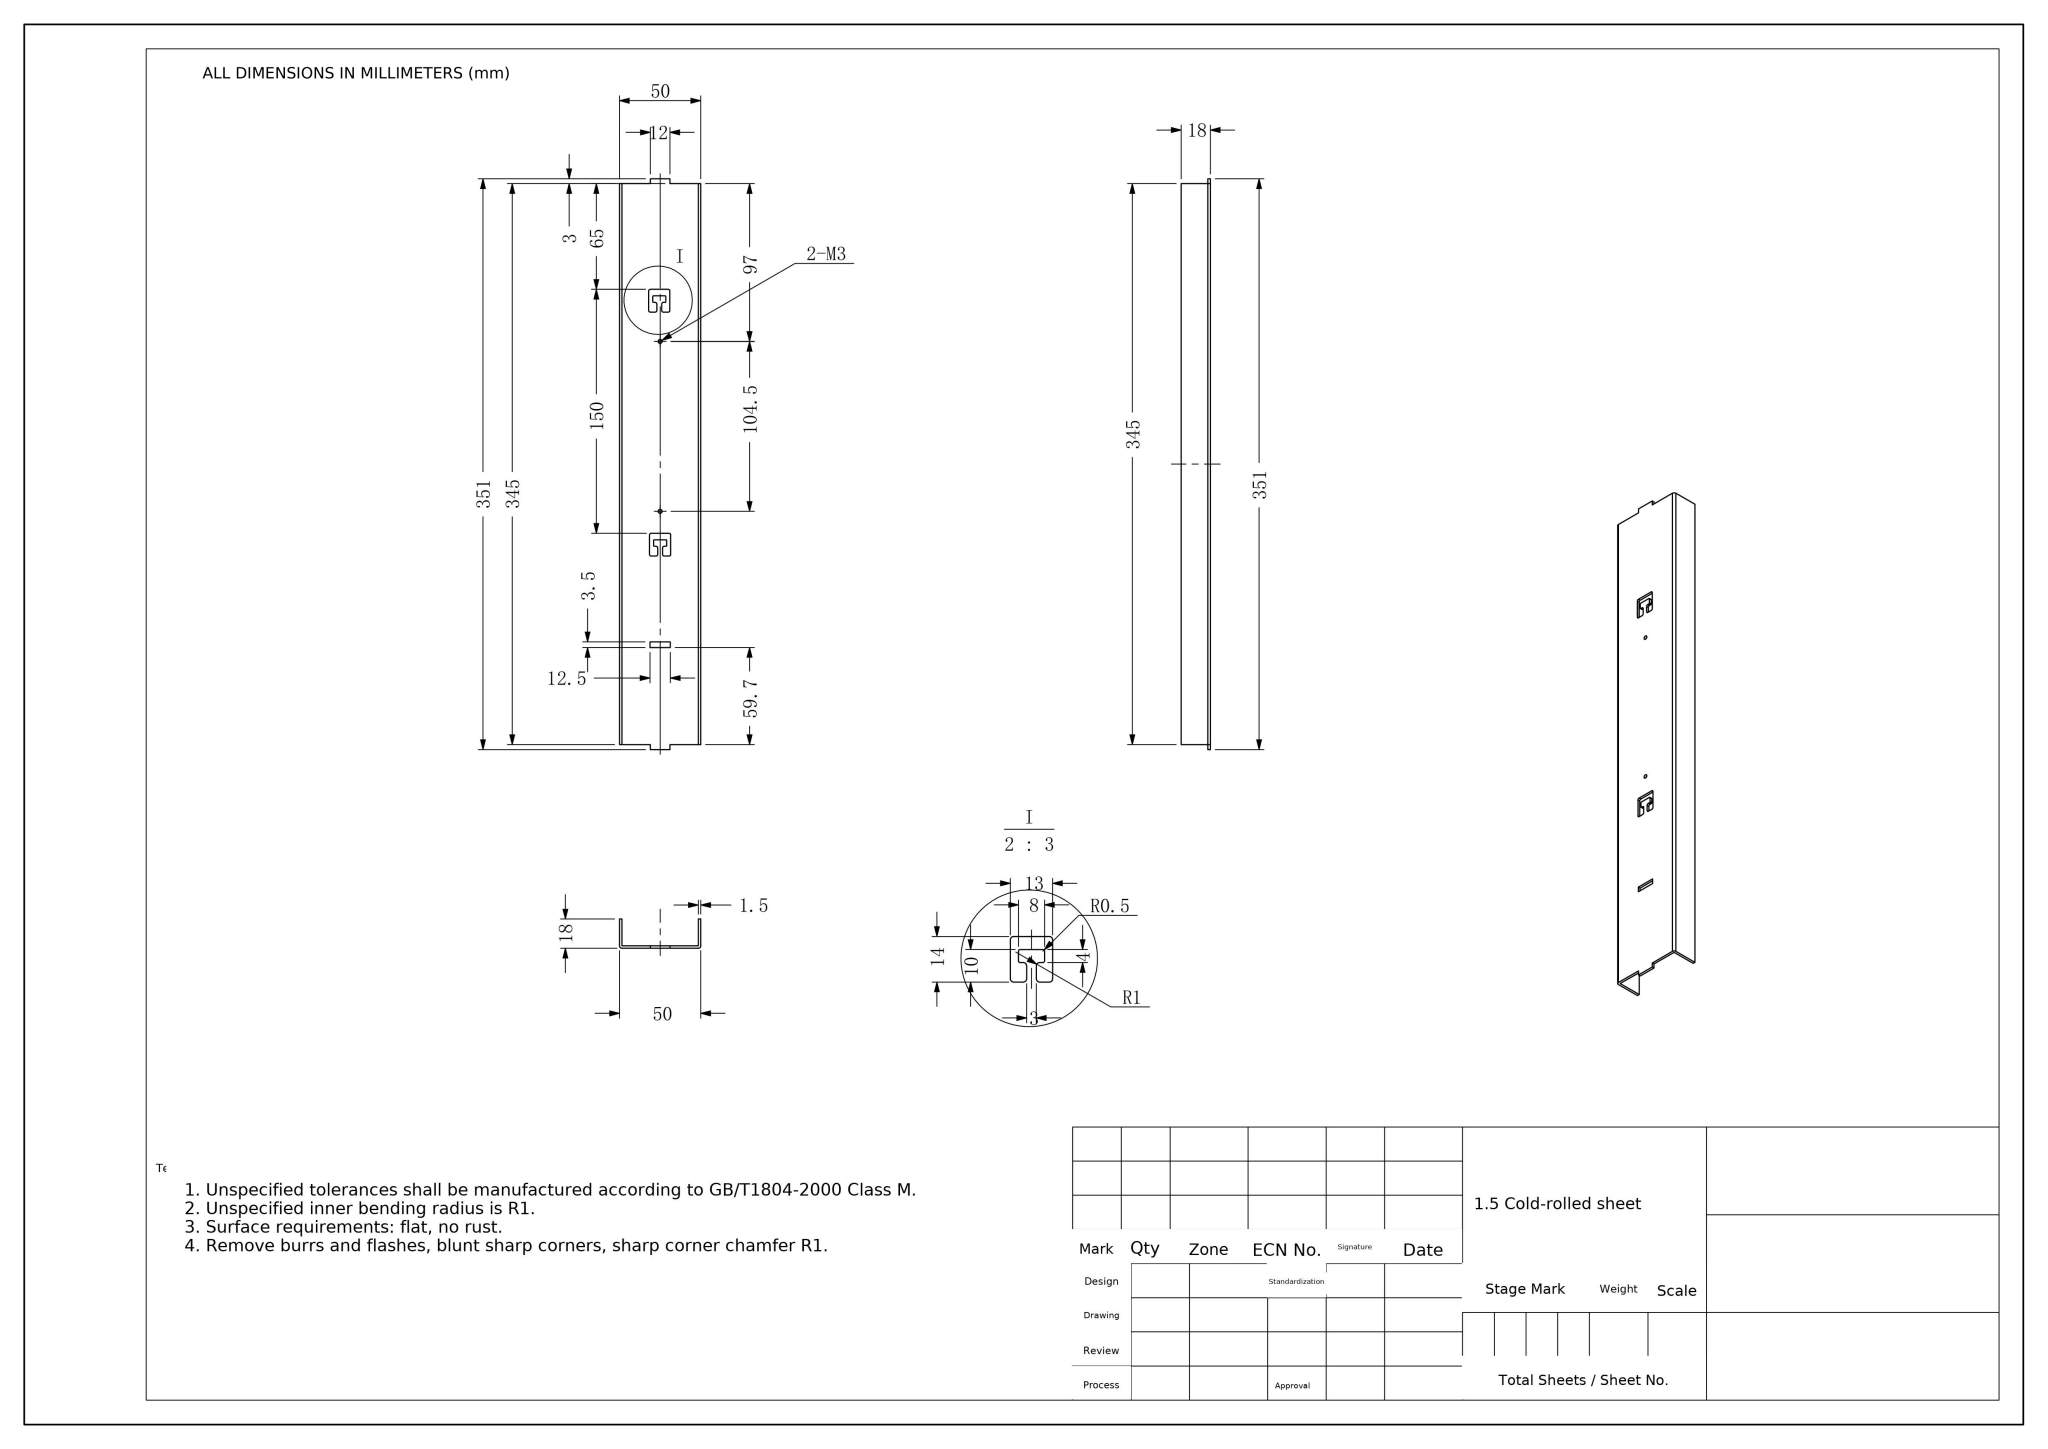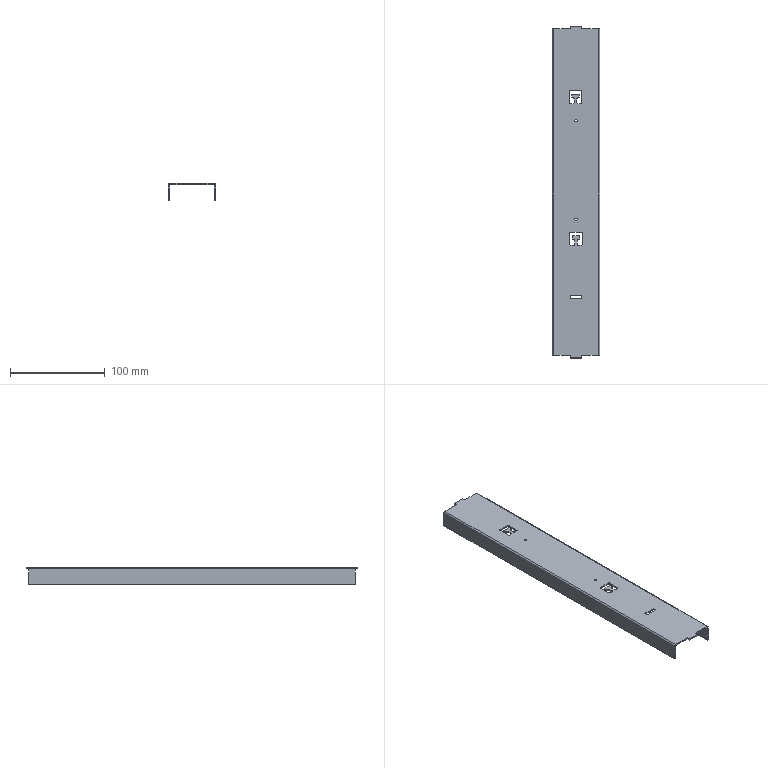Part | NX | mm | 1 solid | 78 faces | box 50 x 351 x 18 mm | volume 42255 mm3 | plane 46 | cylinder 32 | commonest cylinder face diameters 2 x16 1 x8 2.459 x4 0.004 x2 3.004 x2